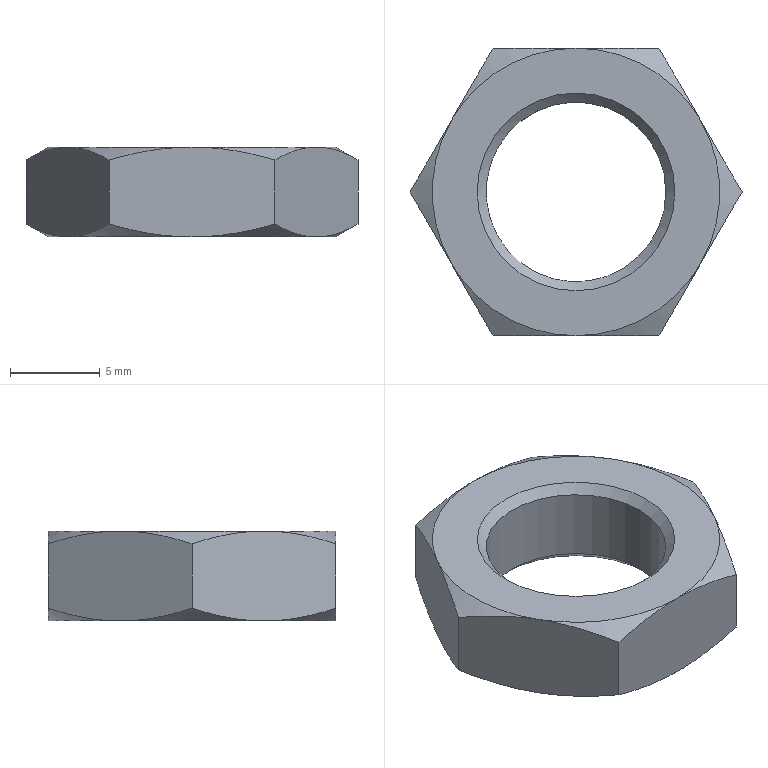Component | NX | GB-T6173-2000_M10X1 | 1 solid | 23 faces | volume 699 mm3 | cone 14 | plane 8 | cylinder 1 | commonest cylinder face diameters 10 x1